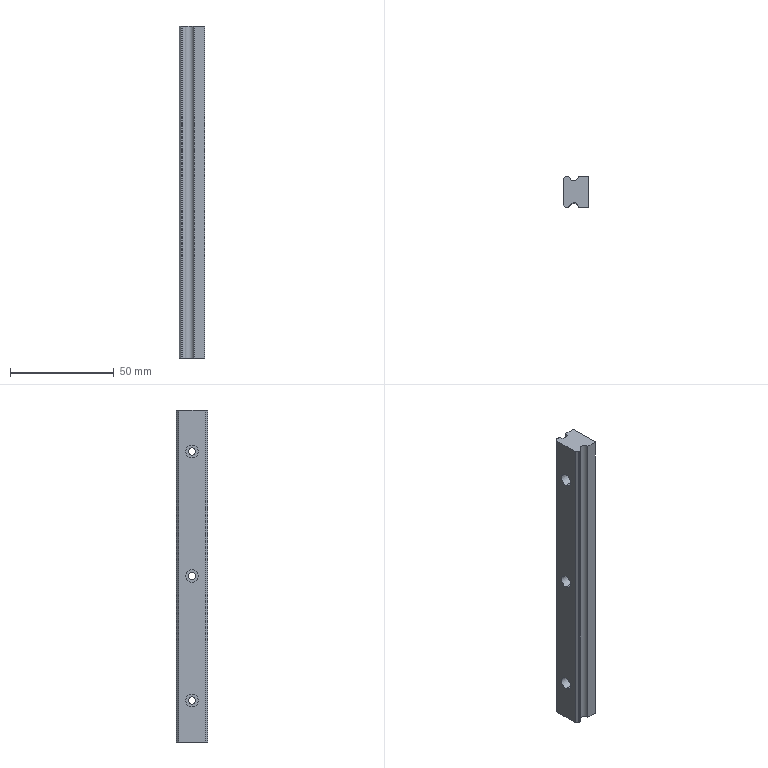Component | SolidWorks | SXRZ24_280-1_LinearGuide-1 | 1 solid | 30 faces | box 12.5 x 15 x 160 mm | volume 26679 mm3 | cylinder 17 | plane 13 | commonest cylinder face diameters 3.5 x6 6 x6 4.4 x3 3 x2
build123d program:
from build123d import *

# Parameters (mm, degrees)
BOSS_EXTRUDE1_DEPTH      = 140
BOSS_EXTRUDE1_DEPTH_BACK = 140
SKETCH7_W                = 125.064
SKETCH7_H                = 80
SKETCH7_W_2              = 316.061
SKETCH7_H_2              = 143.379
CUT_EXTRUDE1_DEPTH       = 141.757


with BuildPart() as part:
    # Sketch1 → Boss-Extrude1 (new, two sides: drawn at the far end of the back side and taken through both)
    with BuildSketch(Plane.XY.offset(-BOSS_EXTRUDE1_DEPTH_BACK)):
        with BuildLine():
            Line((-7.5, 0), (7.5, 0))
            Line((7.5, 0), (7.5, 5.105))
            ThreePointArc((7.5, 5.105), (5.348, 6.849), (6.608, 9.316))
            ThreePointArc((6.608, 9.316), (7.257, 9.869), (7.5, 10.687))
            Line((7.5, 10.687), (7.5, 11.376))
            Line((7.5, 11.376), (6.376, 12.5))
            Line((6.376, 12.5), (-6.376, 12.5))
            Line((-6.376, 12.5), (-7.5, 11.376))
            Line((-7.5, 11.376), (-7.5, 10.687))
            ThreePointArc((-7.5, 10.687), (-7.257, 9.869), (-6.608, 9.316))
            ThreePointArc((-6.608, 9.316), (-5.348, 6.849), (-7.5, 5.105))
            Line((-7.5, 5.105), (-7.5, 0))
        make_face()
    extrude(amount=BOSS_EXTRUDE1_DEPTH + BOSS_EXTRUDE1_DEPTH_BACK)

    # Sketch2 → Cut-Revolve1 (revolve, cut)
    with BuildSketch(Plane(origin=(0, 0, 0), x_dir=(0, 0, -1), z_dir=(1, 0, 0)), mode=Mode.PRIVATE) as cut_revolve1_sk:
        Polygon((120, 12.5), (123, 12.5), (123, 8), (121.75, 8), (121.75, 0), (120, 0), align=None)
    revolve(cut_revolve1_sk.sketch.rotate(Axis((0, 0, -120), (0, 1, 0)), 180), axis=Axis((0, 0, -120), (0, 1, 0)), mode=Mode.SUBTRACT)

    # Sketch3 → Cut-Revolve2 (revolve, cut)
    with BuildSketch(Plane(origin=(0, 0, 0), x_dir=(0, 0, -1), z_dir=(1, 0, 0)), mode=Mode.PRIVATE) as cut_revolve2_sk:
        Polygon((-120, 12.5), (-117, 12.5), (-117, 8), (-118.25, 8), (-118.25, 0), (-120, 0), align=None)
    revolve(cut_revolve2_sk.sketch.rotate(Axis((0, 0, 120), (0, 1, 0)), 180), axis=Axis((0, 0, 120), (0, 1, 0)), mode=Mode.SUBTRACT)

    # Sketch4 → Cut-Revolve3 (revolve, cut)
    with BuildSketch(Plane(origin=(0, 0, 0), x_dir=(0, 0, -1), z_dir=(1, 0, 0)), mode=Mode.PRIVATE) as cut_revolve3_sk:
        Polygon((-60, 12.5), (-57, 12.5), (-57, 8), (-58.25, 8), (-58.25, 0), (-60, 0), align=None)
    revolve(cut_revolve3_sk.sketch.rotate(Axis((0, 0, 60), (0, 1, 0)), 180), axis=Axis((0, 0, 60), (0, 1, 0)), mode=Mode.SUBTRACT)

    # Sketch5 → Cut-Revolve4 (revolve, cut)
    with BuildSketch(Plane(origin=(0, 0, 0), x_dir=(0, 0, -1), z_dir=(1, 0, 0)), mode=Mode.PRIVATE) as cut_revolve4_sk:
        Polygon((0, 12.5), (3, 12.5), (3, 8), (1.75, 8), (1.75, 0), (0, 0), align=None)
    revolve(cut_revolve4_sk.sketch.rotate(Axis((0, 0, 0), (0, 1, 0)), 180), axis=Axis((0, 0, 0), (0, 1, 0)), mode=Mode.SUBTRACT)

    # Sketch6 → Cut-Revolve5 (revolve, cut)
    with BuildSketch(Plane(origin=(0, 0, 0), x_dir=(0, 0, -1), z_dir=(1, 0, 0)), mode=Mode.PRIVATE) as cut_revolve5_sk:
        Polygon((60, 12.5), (63, 12.5), (63, 8), (61.75, 8), (61.75, 0), (60, 0), align=None)
    revolve(cut_revolve5_sk.sketch.rotate(Axis((0, 0, -60), (0, 1, 0)), 180), axis=Axis((0, 0, -60), (0, 1, 0)), mode=Mode.SUBTRACT)

    # Sketch7 → Cut-Extrude1 (cut, through all)
    with BuildSketch(Plane(origin=(0, 12.5, 0), x_dir=(1, 0, 0), z_dir=(0, 1, 0))):
        with Locations((-7.064, 120)):
            Rectangle(SKETCH7_W, SKETCH7_H)
        with Locations((6.803, -151.689)):
            Rectangle(SKETCH7_W_2, SKETCH7_H_2)
    extrude(amount=-CUT_EXTRUDE1_DEPTH, mode=Mode.SUBTRACT)


solid = part.part

# Placed as in the assembly
solid = solid.moved(Location((-772.135, -373.407, 1083.102), (0, 0, 90)))
STEP:
#1=COLOUR_RGB('',0.7922,0.8196,0.9333);
#2=FILL_AREA_STYLE_COLOUR('',#1);
#3=FILL_AREA_STYLE('',(#2));
#4=SURFACE_STYLE_FILL_AREA(#3);
#5=SURFACE_SIDE_STYLE('',(#4));
#6=SURFACE_STYLE_USAGE(.BOTH.,#5);
#7=PRESENTATION_STYLE_ASSIGNMENT((#6));
#8=CARTESIAN_POINT('',(-30.399,-14.701,40.211));
#9=VERTEX_POINT('',#8);
#10=CARTESIAN_POINT('',(-30.399,-14.701,40.349));
#11=VERTEX_POINT('',#10);
#12=CARTESIAN_POINT('',(-30.399,-14.701,40.28));
#13=DIRECTION('',(-1.,-0.,0.));
#14=DIRECTION('',(0.,0.,1.));
#15=AXIS2_PLACEMENT_3D('',#12,#13,#14);
#16=CIRCLE('',#15,0.0689);
#17=EDGE_CURVE('',#9,#11,#16,.T.);
#18=ORIENTED_EDGE('',*,*,#17,.F.);
#19=CARTESIAN_POINT('',(-30.714,-14.701,40.211));
#20=VERTEX_POINT('',#19);
#21=CARTESIAN_POINT('',(-30.399,-14.701,40.211));
#22=DIRECTION('',(-1.,-0.,0.));
#23=VECTOR('',#22,39.37);
#24=LINE('',#21,#23);
#25=EDGE_CURVE('',#9,#20,#24,.T.);
#26=ORIENTED_EDGE('',*,*,#25,.T.);
#27=CARTESIAN_POINT('',(-30.714,-14.701,40.349));
#28=VERTEX_POINT('',#27);
#29=CARTESIAN_POINT('',(-30.714,-14.701,40.28));
#30=DIRECTION('',(-1.,-0.,0.));
#31=DIRECTION('',(0.,0.,1.));
#32=AXIS2_PLACEMENT_3D('',#29,#30,#31);
#33=CIRCLE('',#32,0.0689);
#34=EDGE_CURVE('',#20,#28,#33,.T.);
#35=ORIENTED_EDGE('',*,*,#34,.T.);
#36=CARTESIAN_POINT('',(-30.399,-14.701,40.349));
#37=DIRECTION('',(-1.,-0.,0.));
#38=VECTOR('',#37,39.37);
#39=LINE('',#36,#38);
#40=EDGE_CURVE('',#11,#28,#39,.T.);
#41=ORIENTED_EDGE('',*,*,#40,.F.);
#42=EDGE_LOOP('',(#18,#26,#35,#41));
#43=FACE_OUTER_BOUND('',#42,.T.);
#44=CARTESIAN_POINT('',(-30.399,-14.701,40.28));
#45=DIRECTION('',(-1.,-0.,0.));
#46=DIRECTION('',(0.,0.,1.));
#47=AXIS2_PLACEMENT_3D('',#44,#45,#46);
#48=CYLINDRICAL_SURFACE('',#47,0.0689);
#49=ADVANCED_FACE('',(#43),#48,.F.);
#50=CARTESIAN_POINT('',(-30.714,-14.701,40.161));
#51=VERTEX_POINT('',#50);
#52=CARTESIAN_POINT('',(-30.714,-14.701,40.398));
#53=VERTEX_POINT('',#52);
#54=CARTESIAN_POINT('',(-30.714,-14.701,40.28));
#55=DIRECTION('',(-1.,-0.,0.));
#56=DIRECTION('',(0.,0.,1.));
#57=AXIS2_PLACEMENT_3D('',#54,#55,#56);
#58=CIRCLE('',#57,0.1181);
#59=EDGE_CURVE('',#51,#53,#58,.T.);
#60=ORIENTED_EDGE('',*,*,#59,.F.);
#61=CARTESIAN_POINT('',(-30.891,-14.701,40.161));
#62=VERTEX_POINT('',#61);
#63=CARTESIAN_POINT('',(-30.399,-14.701,40.161));
#64=DIRECTION('',(-1.,-0.,0.));
#65=VECTOR('',#64,39.37);
#66=LINE('',#63,#65);
#67=EDGE_CURVE('',#51,#62,#66,.T.);
#68=ORIENTED_EDGE('',*,*,#67,.T.);
#69=CARTESIAN_POINT('',(-30.891,-14.701,40.398));
#70=VERTEX_POINT('',#69);
#71=CARTESIAN_POINT('',(-30.891,-14.701,40.28));
#72=DIRECTION('',(-1.,-0.,0.));
#73=DIRECTION('',(0.,0.,1.));
#74=AXIS2_PLACEMENT_3D('',#71,#72,#73);
#75=CIRCLE('',#74,0.1181);
#76=EDGE_CURVE('',#62,#70,#75,.T.);
#77=ORIENTED_EDGE('',*,*,#76,.T.);
#78=CARTESIAN_POINT('',(-30.399,-14.701,40.398));
#79=DIRECTION('',(-1.,-0.,0.));
#80=VECTOR('',#79,39.37);
#81=LINE('',#78,#80);
#82=EDGE_CURVE('',#53,#70,#81,.T.);
#83=ORIENTED_EDGE('',*,*,#82,.F.);
#84=EDGE_LOOP('',(#60,#68,#77,#83));
#85=FACE_OUTER_BOUND('',#84,.T.);
#86=CARTESIAN_POINT('',(-30.399,-14.701,40.28));
#87=DIRECTION('',(-1.,-0.,0.));
#88=DIRECTION('',(0.,0.,1.));
#89=AXIS2_PLACEMENT_3D('',#86,#87,#88);
#90=CYLINDRICAL_SURFACE('',#89,0.1181);
#91=ADVANCED_FACE('',(#85),#90,.F.);
#92=CARTESIAN_POINT('',(-30.399,-14.701,42.573));
#93=VERTEX_POINT('',#92);
#94=CARTESIAN_POINT('',(-30.399,-14.701,42.711));
#95=VERTEX_POINT('',#94);
#96=CARTESIAN_POINT('',(-30.399,-14.701,42.642));
#97=DIRECTION('',(-1.,-0.,0.));
#98=DIRECTION('',(0.,0.,1.));
#99=AXIS2_PLACEMENT_3D('',#96,#97,#98);
#100=CIRCLE('',#99,0.0689);
#101=EDGE_CURVE('',#93,#95,#100,.T.);
#102=ORIENTED_EDGE('',*,*,#101,.F.);
#103=CARTESIAN_POINT('',(-30.714,-14.701,42.573));
#104=VERTEX_POINT('',#103);
#105=CARTESIAN_POINT('',(-30.399,-14.701,42.573));
#106=DIRECTION('',(-1.,-0.,0.));
#107=VECTOR('',#106,39.37);
#108=LINE('',#105,#107);
#109=EDGE_CURVE('',#93,#104,#108,.T.);
#110=ORIENTED_EDGE('',*,*,#109,.T.);
#111=CARTESIAN_POINT('',(-30.714,-14.701,42.711));
#112=VERTEX_POINT('',#111);
#113=CARTESIAN_POINT('',(-30.714,-14.701,42.642));
#114=DIRECTION('',(-1.,-0.,0.));
#115=DIRECTION('',(0.,0.,1.));
#116=AXIS2_PLACEMENT_3D('',#113,#114,#115);
#117=CIRCLE('',#116,0.0689);
#118=EDGE_CURVE('',#104,#112,#117,.T.);
#119=ORIENTED_EDGE('',*,*,#118,.T.);
#120=CARTESIAN_POINT('',(-30.399,-14.701,42.711));
#121=DIRECTION('',(-1.,-0.,0.));
#122=VECTOR('',#121,39.37);
#123=LINE('',#120,#122);
#124=EDGE_CURVE('',#95,#112,#123,.T.);
#125=ORIENTED_EDGE('',*,*,#124,.F.);
#126=EDGE_LOOP('',(#102,#110,#119,#125));
#127=FACE_OUTER_BOUND('',#126,.T.);
#128=CARTESIAN_POINT('',(-30.399,-14.701,42.642));
#129=DIRECTION('',(-1.,-0.,0.));
#130=DIRECTION('',(0.,0.,1.));
#131=AXIS2_PLACEMENT_3D('',#128,#129,#130);
#132=CYLINDRICAL_SURFACE('',#131,0.0689);
#133=ADVANCED_FACE('',(#127),#132,.F.);
#134=CARTESIAN_POINT('',(-30.714,-14.701,42.524));
#135=VERTEX_POINT('',#134);
#136=CARTESIAN_POINT('',(-30.714,-14.701,42.76));
#137=VERTEX_POINT('',#136);
#138=CARTESIAN_POINT('',(-30.714,-14.701,42.642));
#139=DIRECTION('',(-1.,-0.,0.));
#140=DIRECTION('',(0.,0.,1.));
#141=AXIS2_PLACEMENT_3D('',#138,#139,#140);
#142=CIRCLE('',#141,0.1181);
#143=EDGE_CURVE('',#135,#137,#142,.T.);
#144=ORIENTED_EDGE('',*,*,#143,.F.);
#145=CARTESIAN_POINT('',(-30.891,-14.701,42.524));
#146=VERTEX_POINT('',#145);
#147=CARTESIAN_POINT('',(-30.399,-14.701,42.524));
#148=DIRECTION('',(-1.,-0.,0.));
#149=VECTOR('',#148,39.37);
#150=LINE('',#147,#149);
#151=EDGE_CURVE('',#135,#146,#150,.T.);
#152=ORIENTED_EDGE('',*,*,#151,.T.);
#153=CARTESIAN_POINT('',(-30.891,-14.701,42.76));
#154=VERTEX_POINT('',#153);
#155=CARTESIAN_POINT('',(-30.891,-14.701,42.642));
#156=DIRECTION('',(-1.,-0.,0.));
#157=DIRECTION('',(0.,0.,1.));
#158=AXIS2_PLACEMENT_3D('',#155,#156,#157);
#159=CIRCLE('',#158,0.1181);
#160=EDGE_CURVE('',#146,#154,#159,.T.);
#161=ORIENTED_EDGE('',*,*,#160,.T.);
#162=CARTESIAN_POINT('',(-30.399,-14.701,42.76));
#163=DIRECTION('',(-1.,-0.,0.));
#164=VECTOR('',#163,39.37);
#165=LINE('',#162,#164);
#166=EDGE_CURVE('',#137,#154,#165,.T.);
#167=ORIENTED_EDGE('',*,*,#166,.F.);
#168=EDGE_LOOP('',(#144,#152,#161,#167));
#169=FACE_OUTER_BOUND('',#168,.T.);
#170=CARTESIAN_POINT('',(-30.399,-14.701,42.642));
#171=DIRECTION('',(-1.,-0.,0.));
#172=DIRECTION('',(0.,0.,1.));
#173=AXIS2_PLACEMENT_3D('',#170,#171,#172);
#174=CYLINDRICAL_SURFACE('',#173,0.1181);
#175=ADVANCED_FACE('',(#169),#174,.F.);
#176=CARTESIAN_POINT('',(-30.399,-14.701,44.935));
#177=VERTEX_POINT('',#176);
#178=CARTESIAN_POINT('',(-30.399,-14.701,45.073));
#179=VERTEX_POINT('',#178);
#180=CARTESIAN_POINT('',(-30.399,-14.701,45.004));
#181=DIRECTION('',(-1.,-0.,0.));
#182=DIRECTION('',(0.,0.,1.));
#183=AXIS2_PLACEMENT_3D('',#180,#181,#182);
#184=CIRCLE('',#183,0.0689);
#185=EDGE_CURVE('',#177,#179,#184,.T.);
#186=ORIENTED_EDGE('',*,*,#185,.F.);
#187=CARTESIAN_POINT('',(-30.714,-14.701,44.935));
#188=VERTEX_POINT('',#187);
#189=CARTESIAN_POINT('',(-30.399,-14.701,44.935));
#190=DIRECTION('',(-1.,-0.,0.));
#191=VECTOR('',#190,39.37);
#192=LINE('',#189,#191);
#193=EDGE_CURVE('',#177,#188,#192,.T.);
#194=ORIENTED_EDGE('',*,*,#193,.T.);
#195=CARTESIAN_POINT('',(-30.714,-14.701,45.073));
#196=VERTEX_POINT('',#195);
#197=CARTESIAN_POINT('',(-30.714,-14.701,45.004));
#198=DIRECTION('',(-1.,-0.,0.));
#199=DIRECTION('',(0.,0.,1.));
#200=AXIS2_PLACEMENT_3D('',#197,#198,#199);
#201=CIRCLE('',#200,0.0689);
#202=EDGE_CURVE('',#188,#196,#201,.T.);
#203=ORIENTED_EDGE('',*,*,#202,.T.);
#204=CARTESIAN_POINT('',(-30.399,-14.701,45.073));
#205=DIRECTION('',(-1.,-0.,0.));
#206=VECTOR('',#205,39.37);
#207=LINE('',#204,#206);
#208=EDGE_CURVE('',#179,#196,#207,.T.);
#209=ORIENTED_EDGE('',*,*,#208,.F.);
#210=EDGE_LOOP('',(#186,#194,#203,#209));
#211=FACE_OUTER_BOUND('',#210,.T.);
#212=CARTESIAN_POINT('',(-30.399,-14.701,45.004));
#213=DIRECTION('',(-1.,-0.,0.));
#214=DIRECTION('',(0.,0.,1.));
#215=AXIS2_PLACEMENT_3D('',#212,#213,#214);
#216=CYLINDRICAL_SURFACE('',#215,0.0689);
#217=ADVANCED_FACE('',(#211),#216,.F.);
#218=CARTESIAN_POINT('',(-30.714,-14.701,44.886));
#219=VERTEX_POINT('',#218);
#220=CARTESIAN_POINT('',(-30.714,-14.701,45.122));
#221=VERTEX_POINT('',#220);
#222=CARTESIAN_POINT('',(-30.714,-14.701,45.004));
#223=DIRECTION('',(-1.,-0.,0.));
#224=DIRECTION('',(0.,0.,1.));
#225=AXIS2_PLACEMENT_3D('',#222,#223,#224);
#226=CIRCLE('',#225,0.1181);
#227=EDGE_CURVE('',#219,#221,#226,.T.);
#228=ORIENTED_EDGE('',*,*,#227,.F.);
#229=CARTESIAN_POINT('',(-30.891,-14.701,44.886));
#230=VERTEX_POINT('',#229);
#231=CARTESIAN_POINT('',(-30.399,-14.701,44.886));
#232=DIRECTION('',(-1.,-0.,0.));
#233=VECTOR('',#232,39.37);
#234=LINE('',#231,#233);
#235=EDGE_CURVE('',#219,#230,#234,.T.);
#236=ORIENTED_EDGE('',*,*,#235,.T.);
#237=CARTESIAN_POINT('',(-30.891,-14.701,45.122));
#238=VERTEX_POINT('',#237);
#239=CARTESIAN_POINT('',(-30.891,-14.701,45.004));
#240=DIRECTION('',(-1.,-0.,0.));
#241=DIRECTION('',(0.,0.,1.));
#242=AXIS2_PLACEMENT_3D('',#239,#240,#241);
#243=CIRCLE('',#242,0.1181);
#244=EDGE_CURVE('',#230,#238,#243,.T.);
#245=ORIENTED_EDGE('',*,*,#244,.T.);
#246=CARTESIAN_POINT('',(-30.399,-14.701,45.122));
#247=DIRECTION('',(-1.,-0.,0.));
#248=VECTOR('',#247,39.37);
#249=LINE('',#246,#248);
#250=EDGE_CURVE('',#221,#238,#249,.T.);
#251=ORIENTED_EDGE('',*,*,#250,.F.);
#252=EDGE_LOOP('',(#228,#236,#245,#251));
#253=FACE_OUTER_BOUND('',#252,.T.);
#254=CARTESIAN_POINT('',(-30.399,-14.701,45.004));
#255=DIRECTION('',(-1.,-0.,0.));
#256=DIRECTION('',(0.,0.,1.));
#257=AXIS2_PLACEMENT_3D('',#254,#255,#256);
#258=CYLINDRICAL_SURFACE('',#257,0.1181);
#259=ADVANCED_FACE('',(#253),#258,.F.);
#260=CARTESIAN_POINT('',(-30.766,-14.441,45.791));
#261=VERTEX_POINT('',#260);
#262=CARTESIAN_POINT('',(-30.687,-14.492,45.791));
#263=VERTEX_POINT('',#262);
#264=CARTESIAN_POINT('',(-30.687,-14.406,45.791));
#265=DIRECTION('',(0.,-0.,1.));
#266=DIRECTION('',(0.,-1.,0.));
#267=AXIS2_PLACEMENT_3D('',#264,#265,#266);
#268=CIRCLE('',#267,0.08661);
#269=EDGE_CURVE('',#261,#263,#268,.T.);
#270=ORIENTED_EDGE('',*,*,#269,.T.);
#271=CARTESIAN_POINT('',(-30.687,-14.492,39.492));
#272=VERTEX_POINT('',#271);
#273=CARTESIAN_POINT('',(-30.687,-14.492,48.154));
#274=DIRECTION('',(-0.,0.,-1.));
#275=VECTOR('',#274,39.37);
#276=LINE('',#273,#275);
#277=EDGE_CURVE('',#263,#272,#276,.T.);
#278=ORIENTED_EDGE('',*,*,#277,.T.);
#279=CARTESIAN_POINT('',(-30.766,-14.441,39.492));
#280=VERTEX_POINT('',#279);
#281=CARTESIAN_POINT('',(-30.687,-14.406,39.492));
#282=DIRECTION('',(-0.,0.,-1.));
#283=DIRECTION('',(0.,1.,0.));
#284=AXIS2_PLACEMENT_3D('',#281,#282,#283);
#285=CIRCLE('',#284,0.08661);
#286=EDGE_CURVE('',#272,#280,#285,.T.);
#287=ORIENTED_EDGE('',*,*,#286,.T.);
#288=CARTESIAN_POINT('',(-30.766,-14.441,48.154));
#289=DIRECTION('',(-0.,0.,-1.));
#290=VECTOR('',#289,39.37);
#291=LINE('',#288,#290);
#292=EDGE_CURVE('',#261,#280,#291,.T.);
#293=ORIENTED_EDGE('',*,*,#292,.F.);
#294=EDGE_LOOP('',(#270,#278,#287,#293));
#295=FACE_OUTER_BOUND('',#294,.T.);
#296=CARTESIAN_POINT('',(-30.687,-14.406,48.154));
#297=DIRECTION('',(-0.,0.,-1.));
#298=DIRECTION('',(0.,-1.,0.));
#299=AXIS2_PLACEMENT_3D('',#296,#297,#298);
#300=CYLINDRICAL_SURFACE('',#299,0.08661);
#301=ADVANCED_FACE('',(#295),#300,.F.);
#302=CARTESIAN_POINT('',(-30.399,-14.701,42.642));
#303=DIRECTION('',(-1.,-0.,0.));
#304=DIRECTION('',(0.,0.,1.));
#305=AXIS2_PLACEMENT_3D('',#302,#303,#304);
#306=CIRCLE('',#305,0.0689);
#307=EDGE_CURVE('',#95,#93,#306,.T.);
#308=ORIENTED_EDGE('',*,*,#307,.T.);
#309=ORIENTED_EDGE('',*,*,#101,.T.);
#310=EDGE_LOOP('',(#308,#309));
#311=FACE_BOUND('',#310,.T.);
#312=CARTESIAN_POINT('',(-30.399,-14.406,45.791));
#313=VERTEX_POINT('',#312);
#314=CARTESIAN_POINT('',(-30.399,-14.406,39.492));
#315=VERTEX_POINT('',#314);
#316=CARTESIAN_POINT('',(-30.399,-14.406,48.154));
#317=DIRECTION('',(-0.,0.,-1.));
#318=VECTOR('',#317,39.37);
#319=LINE('',#316,#318);
#320=EDGE_CURVE('',#313,#315,#319,.T.);
#321=ORIENTED_EDGE('',*,*,#320,.F.);
#322=CARTESIAN_POINT('',(-30.399,-14.996,45.791));
#323=VERTEX_POINT('',#322);
#324=CARTESIAN_POINT('',(-30.399,-20.655,45.791));
#325=DIRECTION('',(0.,-1.,-0.));
#326=VECTOR('',#325,39.37);
#327=LINE('',#324,#326);
#328=EDGE_CURVE('',#313,#323,#327,.T.);
#329=ORIENTED_EDGE('',*,*,#328,.T.);
#330=CARTESIAN_POINT('',(-30.399,-14.996,39.492));
#331=VERTEX_POINT('',#330);
#332=CARTESIAN_POINT('',(-30.399,-14.996,48.154));
#333=DIRECTION('',(-0.,0.,-1.));
#334=VECTOR('',#333,39.37);
#335=LINE('',#332,#334);
#336=EDGE_CURVE('',#323,#331,#335,.T.);
#337=ORIENTED_EDGE('',*,*,#336,.T.);
#338=CARTESIAN_POINT('',(-30.399,-17.441,39.492));
#339=DIRECTION('',(-0.,1.,0.));
#340=VECTOR('',#339,39.37);
#341=LINE('',#338,#340);
#342=EDGE_CURVE('',#331,#315,#341,.T.);
#343=ORIENTED_EDGE('',*,*,#342,.T.);
#344=EDGE_LOOP('',(#321,#329,#337,#343));
#345=FACE_OUTER_BOUND('',#344,.T.);
#346=CARTESIAN_POINT('',(-30.399,-14.701,45.004));
#347=DIRECTION('',(-1.,-0.,0.));
#348=DIRECTION('',(0.,0.,1.));
#349=AXIS2_PLACEMENT_3D('',#346,#347,#348);
#350=CIRCLE('',#349,0.0689);
#351=EDGE_CURVE('',#179,#177,#350,.T.);
#352=ORIENTED_EDGE('',*,*,#351,.T.);
#353=ORIENTED_EDGE('',*,*,#185,.T.);
#354=EDGE_LOOP('',(#352,#353));
#355=FACE_BOUND('',#354,.T.);
#356=CARTESIAN_POINT('',(-30.399,-14.701,40.28));
#357=DIRECTION('',(-1.,-0.,0.));
#358=DIRECTION('',(0.,0.,1.));
#359=AXIS2_PLACEMENT_3D('',#356,#357,#358);
#360=CIRCLE('',#359,0.0689);
#361=EDGE_CURVE('',#11,#9,#360,.T.);
#362=ORIENTED_EDGE('',*,*,#361,.T.);
#363=ORIENTED_EDGE('',*,*,#17,.T.);
#364=EDGE_LOOP('',(#362,#363));
#365=FACE_BOUND('',#364,.T.);
#366=CARTESIAN_POINT('',(-30.399,-14.996,48.154));
#367=DIRECTION('',(-1.,-0.,0.));
#368=DIRECTION('',(0.,-0.,1.));
#369=AXIS2_PLACEMENT_3D('',#366,#367,#368);
#370=PLANE('',#369);
#371=ADVANCED_FACE('',(#311,#345,#355,#365),#370,.F.);
#372=CARTESIAN_POINT('',(-30.891,-14.701,42.642));
#373=DIRECTION('',(-1.,-0.,0.));
#374=DIRECTION('',(0.,0.,1.));
#375=AXIS2_PLACEMENT_3D('',#372,#373,#374);
#376=CIRCLE('',#375,0.1181);
#377=EDGE_CURVE('',#154,#146,#376,.T.);
#378=ORIENTED_EDGE('',*,*,#377,.F.);
#379=ORIENTED_EDGE('',*,*,#160,.F.);
#380=EDGE_LOOP('',(#378,#379));
#381=FACE_BOUND('',#380,.T.);
#382=CARTESIAN_POINT('',(-30.891,-14.952,45.791));
#383=VERTEX_POINT('',#382);
#384=CARTESIAN_POINT('',(-30.891,-14.952,39.492));
#385=VERTEX_POINT('',#384);
#386=CARTESIAN_POINT('',(-30.891,-14.952,48.154));
#387=DIRECTION('',(-0.,0.,-1.));
#388=VECTOR('',#387,39.37);
#389=LINE('',#386,#388);
#390=EDGE_CURVE('',#383,#385,#389,.T.);
#391=ORIENTED_EDGE('',*,*,#390,.F.);
#392=CARTESIAN_POINT('',(-30.891,-14.45,45.791));
#393=VERTEX_POINT('',#392);
#394=CARTESIAN_POINT('',(-30.891,-20.655,45.791));
#395=DIRECTION('',(0.,-1.,-0.));
#396=VECTOR('',#395,39.37);
#397=LINE('',#394,#396);
#398=EDGE_CURVE('',#393,#383,#397,.T.);
#399=ORIENTED_EDGE('',*,*,#398,.F.);
#400=CARTESIAN_POINT('',(-30.891,-14.45,39.492));
#401=VERTEX_POINT('',#400);
#402=CARTESIAN_POINT('',(-30.891,-14.45,48.154));
#403=DIRECTION('',(-0.,0.,-1.));
#404=VECTOR('',#403,39.37);
#405=LINE('',#402,#404);
#406=EDGE_CURVE('',#393,#401,#405,.T.);
#407=ORIENTED_EDGE('',*,*,#406,.T.);
#408=CARTESIAN_POINT('',(-30.891,-17.441,39.492));
#409=DIRECTION('',(-0.,1.,0.));
#410=VECTOR('',#409,39.37);
#411=LINE('',#408,#410);
#412=EDGE_CURVE('',#385,#401,#411,.T.);
#413=ORIENTED_EDGE('',*,*,#412,.F.);
#414=EDGE_LOOP('',(#391,#399,#407,#413));
#415=FACE_OUTER_BOUND('',#414,.T.);
#416=CARTESIAN_POINT('',(-30.891,-14.701,45.004));
#417=DIRECTION('',(-1.,-0.,0.));
#418=DIRECTION('',(0.,0.,1.));
#419=AXIS2_PLACEMENT_3D('',#416,#417,#418);
#420=CIRCLE('',#419,0.1181);
#421=EDGE_CURVE('',#238,#230,#420,.T.);
#422=ORIENTED_EDGE('',*,*,#421,.F.);
#423=ORIENTED_EDGE('',*,*,#244,.F.);
#424=EDGE_LOOP('',(#422,#423));
#425=FACE_BOUND('',#424,.T.);
#426=CARTESIAN_POINT('',(-30.891,-14.701,40.28));
#427=DIRECTION('',(-1.,-0.,0.));
#428=DIRECTION('',(0.,0.,1.));
#429=AXIS2_PLACEMENT_3D('',#426,#427,#428);
#430=CIRCLE('',#429,0.1181);
#431=EDGE_CURVE('',#70,#62,#430,.T.);
#432=ORIENTED_EDGE('',*,*,#431,.F.);
#433=ORIENTED_EDGE('',*,*,#76,.F.);
#434=EDGE_LOOP('',(#432,#433));
#435=FACE_BOUND('',#434,.T.);
#436=CARTESIAN_POINT('',(-30.891,-14.45,48.154));
#437=DIRECTION('',(1.,0.,-0.));
#438=DIRECTION('',(-0.,0.,-1.));
#439=AXIS2_PLACEMENT_3D('',#436,#437,#438);
#440=PLANE('',#439);
#441=ADVANCED_FACE('',(#381,#415,#425,#435),#440,.F.);
#442=ORIENTED_EDGE('',*,*,#336,.F.);
#443=CARTESIAN_POINT('',(-30.6,-14.996,45.791));
#444=VERTEX_POINT('',#443);
#445=CARTESIAN_POINT('',(-30.6,-14.996,45.791));
#446=DIRECTION('',(-1.,-0.,0.));
#447=VECTOR('',#446,39.37);
#448=LINE('',#445,#447);
#449=EDGE_CURVE('',#323,#444,#448,.T.);
#450=ORIENTED_EDGE('',*,*,#449,.T.);
#451=CARTESIAN_POINT('',(-30.6,-14.996,39.492));
#452=VERTEX_POINT('',#451);
#453=CARTESIAN_POINT('',(-30.6,-14.996,48.154));
#454=DIRECTION('',(-0.,0.,-1.));
#455=VECTOR('',#454,39.37);
#456=LINE('',#453,#455);
#457=EDGE_CURVE('',#444,#452,#456,.T.);
#458=ORIENTED_EDGE('',*,*,#457,.T.);
#459=CARTESIAN_POINT('',(-30.6,-14.996,39.492));
#460=DIRECTION('',(1.,0.,-0.));
#461=VECTOR('',#460,39.37);
#462=LINE('',#459,#461);
#463=EDGE_CURVE('',#452,#331,#462,.T.);
#464=ORIENTED_EDGE('',*,*,#463,.T.);
#465=EDGE_LOOP('',(#442,#450,#458,#464));
#466=FACE_OUTER_BOUND('',#465,.T.);
#467=CARTESIAN_POINT('',(-30.6,-14.996,48.154));
#468=DIRECTION('',(-0.,1.,0.));
#469=DIRECTION('',(-0.,0.,-1.));
#470=AXIS2_PLACEMENT_3D('',#467,#468,#469);
#471=PLANE('',#470);
#472=ADVANCED_FACE('',(#466),#471,.F.);
#473=CARTESIAN_POINT('',(-30.6,-14.406,45.791));
#474=VERTEX_POINT('',#473);
#475=CARTESIAN_POINT('',(-30.6,-14.406,39.492));
#476=VERTEX_POINT('',#475);
#477=CARTESIAN_POINT('',(-30.6,-14.406,48.154));
#478=DIRECTION('',(-0.,0.,-1.));
#479=VECTOR('',#478,39.37);
#480=LINE('',#477,#479);
#481=EDGE_CURVE('',#474,#476,#480,.T.);
#482=ORIENTED_EDGE('',*,*,#481,.F.);
#483=CARTESIAN_POINT('',(-30.399,-14.406,45.791));
#484=DIRECTION('',(1.,0.,-0.));
#485=VECTOR('',#484,39.37);
#486=LINE('',#483,#485);
#487=EDGE_CURVE('',#474,#313,#486,.T.);
#488=ORIENTED_EDGE('',*,*,#487,.T.);
#489=ORIENTED_EDGE('',*,*,#320,.T.);
#490=CARTESIAN_POINT('',(-30.399,-14.406,39.492));
#491=DIRECTION('',(-1.,-0.,0.));
#492=VECTOR('',#491,39.37);
#493=LINE('',#490,#492);
#494=EDGE_CURVE('',#315,#476,#493,.T.);
#495=ORIENTED_EDGE('',*,*,#494,.T.);
#496=EDGE_LOOP('',(#482,#488,#489,#495));
#497=FACE_OUTER_BOUND('',#496,.T.);
#498=CARTESIAN_POINT('',(-30.399,-14.406,48.154));
#499=DIRECTION('',(0.,-1.,-0.));
#500=DIRECTION('',(0.,-0.,1.));
#501=AXIS2_PLACEMENT_3D('',#498,#499,#500);
#502=PLANE('',#501);
#503=ADVANCED_FACE('',(#497),#502,.F.);
#504=ORIENTED_EDGE('',*,*,#277,.F.);
#505=CARTESIAN_POINT('',(-30.687,-14.406,45.791));
#506=DIRECTION('',(0.,-0.,1.));
#507=DIRECTION('',(0.,-1.,0.));
#508=AXIS2_PLACEMENT_3D('',#505,#506,#507);
#509=CIRCLE('',#508,0.08661);
#510=EDGE_CURVE('',#263,#474,#509,.T.);
#511=ORIENTED_EDGE('',*,*,#510,.T.);
#512=ORIENTED_EDGE('',*,*,#481,.T.);
#513=CARTESIAN_POINT('',(-30.687,-14.406,39.492));
#514=DIRECTION('',(-0.,0.,-1.));
#515=DIRECTION('',(0.,1.,0.));
#516=AXIS2_PLACEMENT_3D('',#513,#514,#515);
#517=CIRCLE('',#516,0.08661);
#518=EDGE_CURVE('',#476,#272,#517,.T.);
#519=ORIENTED_EDGE('',*,*,#518,.T.);
#520=EDGE_LOOP('',(#504,#511,#512,#519));
#521=FACE_OUTER_BOUND('',#520,.T.);
#522=CARTESIAN_POINT('',(-30.687,-14.406,48.154));
#523=DIRECTION('',(-0.,0.,-1.));
#524=DIRECTION('',(0.,-1.,0.));
#525=AXIS2_PLACEMENT_3D('',#522,#523,#524);
#526=CYLINDRICAL_SURFACE('',#525,0.08661);
#527=ADVANCED_FACE('',(#521),#526,.F.);
#528=CARTESIAN_POINT('',(-30.82,-14.406,45.791));
#529=VERTEX_POINT('',#528);
#530=CARTESIAN_POINT('',(-30.82,-14.406,39.492));
#531=VERTEX_POINT('',#530);
#532=CARTESIAN_POINT('',(-30.82,-14.406,48.154));
#533=DIRECTION('',(-0.,0.,-1.));
#534=VECTOR('',#533,39.37);
#535=LINE('',#532,#534);
#536=EDGE_CURVE('',#529,#531,#535,.T.);
#537=ORIENTED_EDGE('',*,*,#536,.F.);
#538=CARTESIAN_POINT('',(-30.82,-14.465,45.791));
#539=DIRECTION('',(-0.,0.,-1.));
#540=DIRECTION('',(0.,-1.,0.));
#541=AXIS2_PLACEMENT_3D('',#538,#539,#540);
#542=CIRCLE('',#541,0.05906);
#543=EDGE_CURVE('',#529,#261,#542,.T.);
#544=ORIENTED_EDGE('',*,*,#543,.T.);
#545=ORIENTED_EDGE('',*,*,#292,.T.);
#546=CARTESIAN_POINT('',(-30.82,-14.465,39.492));
#547=DIRECTION('',(0.,-0.,1.));
#548=DIRECTION('',(0.,1.,0.));
#549=AXIS2_PLACEMENT_3D('',#546,#547,#548);
#550=CIRCLE('',#549,0.05906);
#551=EDGE_CURVE('',#280,#531,#550,.T.);
#552=ORIENTED_EDGE('',*,*,#551,.T.);
#553=EDGE_LOOP('',(#537,#544,#545,#552));
#554=FACE_OUTER_BOUND('',#553,.T.);
#555=CARTESIAN_POINT('',(-30.82,-14.465,48.154));
#556=DIRECTION('',(-0.,0.,-1.));
#557=DIRECTION('',(0.,-1.,0.));
#558=AXIS2_PLACEMENT_3D('',#555,#556,#557);
#559=CYLINDRICAL_SURFACE('',#558,0.05906);
#560=ADVANCED_FACE('',(#554),#559,.T.);
#561=CARTESIAN_POINT('',(-30.847,-14.406,45.791));
#562=VERTEX_POINT('',#561);
#563=CARTESIAN_POINT('',(-30.847,-14.406,39.492));
#564=VERTEX_POINT('',#563);
#565=CARTESIAN_POINT('',(-30.847,-14.406,48.154));
#566=DIRECTION('',(-0.,0.,-1.));
#567=VECTOR('',#566,39.37);
#568=LINE('',#565,#567);
#569=EDGE_CURVE('',#562,#564,#568,.T.);
#570=ORIENTED_EDGE('',*,*,#569,.F.);
#571=CARTESIAN_POINT('',(-30.82,-14.406,45.791));
#572=DIRECTION('',(1.,0.,-0.));
#573=VECTOR('',#572,39.37);
#574=LINE('',#571,#573);
#575=EDGE_CURVE('',#562,#529,#574,.T.);
#576=ORIENTED_EDGE('',*,*,#575,.T.);
#577=ORIENTED_EDGE('',*,*,#536,.T.);
#578=CARTESIAN_POINT('',(-30.82,-14.406,39.492));
#579=DIRECTION('',(-1.,-0.,0.));
#580=VECTOR('',#579,39.37);
#581=LINE('',#578,#580);
#582=EDGE_CURVE('',#531,#564,#581,.T.);
#583=ORIENTED_EDGE('',*,*,#582,.T.);
#584=EDGE_LOOP('',(#570,#576,#577,#583));
#585=FACE_OUTER_BOUND('',#584,.T.);
#586=CARTESIAN_POINT('',(-30.82,-14.406,48.154));
#587=DIRECTION('',(0.,-1.,-0.));
#588=DIRECTION('',(0.,-0.,1.));
#589=AXIS2_PLACEMENT_3D('',#586,#587,#588);
#590=PLANE('',#589);
#591=ADVANCED_FACE('',(#585),#590,.F.);
#592=ORIENTED_EDGE('',*,*,#406,.F.);
#593=CARTESIAN_POINT('',(-30.847,-14.406,45.791));
#594=DIRECTION('',(0.7071,0.7071,0.));
#595=VECTOR('',#594,39.37);
#596=LINE('',#593,#595);
#597=EDGE_CURVE('',#393,#562,#596,.T.);
#598=ORIENTED_EDGE('',*,*,#597,.T.);
#599=ORIENTED_EDGE('',*,*,#569,.T.);
#600=CARTESIAN_POINT('',(-30.847,-14.406,39.492));
#601=DIRECTION('',(-0.7071,-0.7071,-0.));
#602=VECTOR('',#601,39.37);
#603=LINE('',#600,#602);
#604=EDGE_CURVE('',#564,#401,#603,.T.);
#605=ORIENTED_EDGE('',*,*,#604,.T.);
#606=EDGE_LOOP('',(#592,#598,#599,#605));
#607=FACE_OUTER_BOUND('',#606,.T.);
#608=CARTESIAN_POINT('',(-30.847,-14.406,48.154));
#609=DIRECTION('',(0.7071,-0.7071,-0.));
#610=DIRECTION('',(0.7071,0.7071,0.));
#611=AXIS2_PLACEMENT_3D('',#608,#609,#610);
#612=PLANE('',#611);
#613=ADVANCED_FACE('',(#607),#612,.F.);
#614=CARTESIAN_POINT('',(-30.847,-14.996,45.791));
#615=VERTEX_POINT('',#614);
#616=CARTESIAN_POINT('',(-30.847,-14.996,39.492));
#617=VERTEX_POINT('',#616);
#618=CARTESIAN_POINT('',(-30.847,-14.996,48.154));
#619=DIRECTION('',(-0.,0.,-1.));
#620=VECTOR('',#619,39.37);
#621=LINE('',#618,#620);
#622=EDGE_CURVE('',#615,#617,#621,.T.);
#623=ORIENTED_EDGE('',*,*,#622,.F.);
#624=CARTESIAN_POINT('',(-30.891,-14.952,45.791));
#625=DIRECTION('',(-0.7071,0.7071,0.));
#626=VECTOR('',#625,39.37);
#627=LINE('',#624,#626);
#628=EDGE_CURVE('',#615,#383,#627,.T.);
#629=ORIENTED_EDGE('',*,*,#628,.T.);
#630=ORIENTED_EDGE('',*,*,#390,.T.);
#631=CARTESIAN_POINT('',(-30.891,-14.952,39.492));
#632=DIRECTION('',(0.7071,-0.7071,-0.));
#633=VECTOR('',#632,39.37);
#634=LINE('',#631,#633);
#635=EDGE_CURVE('',#385,#617,#634,.T.);
#636=ORIENTED_EDGE('',*,*,#635,.T.);
#637=EDGE_LOOP('',(#623,#629,#630,#636));
#638=FACE_OUTER_BOUND('',#637,.T.);
#639=CARTESIAN_POINT('',(-30.891,-14.952,48.154));
#640=DIRECTION('',(0.7071,0.7071,0.));
#641=DIRECTION('',(-0.7071,0.7071,0.));
#642=AXIS2_PLACEMENT_3D('',#639,#640,#641);
#643=PLANE('',#642);
#644=ADVANCED_FACE('',(#638),#643,.F.);
#645=CARTESIAN_POINT('',(-30.82,-14.996,45.791));
#646=VERTEX_POINT('',#645);
#647=CARTESIAN_POINT('',(-30.82,-14.996,39.492));
#648=VERTEX_POINT('',#647);
#649=CARTESIAN_POINT('',(-30.82,-14.996,48.154));
#650=DIRECTION('',(-0.,0.,-1.));
#651=VECTOR('',#650,39.37);
#652=LINE('',#649,#651);
#653=EDGE_CURVE('',#646,#648,#652,.T.);
#654=ORIENTED_EDGE('',*,*,#653,.F.);
#655=CARTESIAN_POINT('',(-30.847,-14.996,45.791));
#656=DIRECTION('',(-1.,-0.,0.));
#657=VECTOR('',#656,39.37);
#658=LINE('',#655,#657);
#659=EDGE_CURVE('',#646,#615,#658,.T.);
#660=ORIENTED_EDGE('',*,*,#659,.T.);
#661=ORIENTED_EDGE('',*,*,#622,.T.);
#662=CARTESIAN_POINT('',(-30.847,-14.996,39.492));
#663=DIRECTION('',(1.,0.,-0.));
#664=VECTOR('',#663,39.37);
#665=LINE('',#662,#664);
#666=EDGE_CURVE('',#617,#648,#665,.T.);
#667=ORIENTED_EDGE('',*,*,#666,.T.);
#668=EDGE_LOOP('',(#654,#660,#661,#667));
#669=FACE_OUTER_BOUND('',#668,.T.);
#670=CARTESIAN_POINT('',(-30.847,-14.996,48.154));
#671=DIRECTION('',(-0.,1.,0.));
#672=DIRECTION('',(-0.,0.,-1.));
#673=AXIS2_PLACEMENT_3D('',#670,#671,#672);
#674=PLANE('',#673);
#675=ADVANCED_FACE('',(#669),#674,.F.);
#676=CARTESIAN_POINT('',(-30.766,-14.961,45.791));
#677=VERTEX_POINT('',#676);
#678=CARTESIAN_POINT('',(-30.766,-14.961,39.492));
#679=VERTEX_POINT('',#678);
#680=CARTESIAN_POINT('',(-30.766,-14.961,48.154));
#681=DIRECTION('',(-0.,0.,-1.));
#682=VECTOR('',#681,39.37);
#683=LINE('',#680,#682);
#684=EDGE_CURVE('',#677,#679,#683,.T.);
#685=ORIENTED_EDGE('',*,*,#684,.F.);
#686=CARTESIAN_POINT('',(-30.82,-14.937,45.791));
#687=DIRECTION('',(-0.,0.,-1.));
#688=DIRECTION('',(0.,-1.,0.));
#689=AXIS2_PLACEMENT_3D('',#686,#687,#688);
#690=CIRCLE('',#689,0.05906);
#691=EDGE_CURVE('',#677,#646,#690,.T.);
#692=ORIENTED_EDGE('',*,*,#691,.T.);
#693=ORIENTED_EDGE('',*,*,#653,.T.);
#694=CARTESIAN_POINT('',(-30.82,-14.937,39.492));
#695=DIRECTION('',(0.,-0.,1.));
#696=DIRECTION('',(0.,1.,0.));
#697=AXIS2_PLACEMENT_3D('',#694,#695,#696);
#698=CIRCLE('',#697,0.05906);
#699=EDGE_CURVE('',#648,#679,#698,.T.);
#700=ORIENTED_EDGE('',*,*,#699,.T.);
#701=EDGE_LOOP('',(#685,#692,#693,#700));
#702=FACE_OUTER_BOUND('',#701,.T.);
#703=CARTESIAN_POINT('',(-30.82,-14.937,48.154));
#704=DIRECTION('',(-0.,0.,-1.));
#705=DIRECTION('',(0.,-1.,0.));
#706=AXIS2_PLACEMENT_3D('',#703,#704,#705);
#707=CYLINDRICAL_SURFACE('',#706,0.05906);
#708=ADVANCED_FACE('',(#702),#707,.T.);
#709=ORIENTED_EDGE('',*,*,#457,.F.);
#710=CARTESIAN_POINT('',(-30.687,-14.996,45.791));
#711=DIRECTION('',(0.,-0.,1.));
#712=DIRECTION('',(0.,-1.,0.));
#713=AXIS2_PLACEMENT_3D('',#710,#711,#712);
#714=CIRCLE('',#713,0.08661);
#715=EDGE_CURVE('',#444,#677,#714,.T.);
#716=ORIENTED_EDGE('',*,*,#715,.T.);
#717=ORIENTED_EDGE('',*,*,#684,.T.);
#718=CARTESIAN_POINT('',(-30.687,-14.996,39.492));
#719=DIRECTION('',(-0.,0.,-1.));
#720=DIRECTION('',(0.,1.,0.));
#721=AXIS2_PLACEMENT_3D('',#718,#719,#720);
#722=CIRCLE('',#721,0.08661);
#723=EDGE_CURVE('',#679,#452,#722,.T.);
#724=ORIENTED_EDGE('',*,*,#723,.T.);
#725=EDGE_LOOP('',(#709,#716,#717,#724));
#726=FACE_OUTER_BOUND('',#725,.T.);
#727=CARTESIAN_POINT('',(-30.687,-14.996,48.154));
#728=DIRECTION('',(-0.,0.,-1.));
#729=DIRECTION('',(0.,-1.,0.));
#730=AXIS2_PLACEMENT_3D('',#727,#728,#729);
#731=CYLINDRICAL_SURFACE('',#730,0.08661);
#732=ADVANCED_FACE('',(#726),#731,.F.);
#733=ORIENTED_EDGE('',*,*,#235,.F.);
#734=CARTESIAN_POINT('',(-30.714,-14.701,45.004));
#735=DIRECTION('',(-1.,-0.,0.));
#736=DIRECTION('',(0.,0.,1.));
#737=AXIS2_PLACEMENT_3D('',#734,#735,#736);
#738=CIRCLE('',#737,0.1181);
#739=EDGE_CURVE('',#221,#219,#738,.T.);
#740=ORIENTED_EDGE('',*,*,#739,.F.);
#741=ORIENTED_EDGE('',*,*,#250,.T.);
#742=ORIENTED_EDGE('',*,*,#421,.T.);
#743=EDGE_LOOP('',(#733,#740,#741,#742));
#744=FACE_OUTER_BOUND('',#743,.T.);
#745=CARTESIAN_POINT('',(-30.399,-14.701,45.004));
#746=DIRECTION('',(-1.,-0.,0.));
#747=DIRECTION('',(0.,0.,1.));
#748=AXIS2_PLACEMENT_3D('',#745,#746,#747);
#749=CYLINDRICAL_SURFACE('',#748,0.1181);
#750=ADVANCED_FACE('',(#744),#749,.F.);
#751=ORIENTED_EDGE('',*,*,#739,.T.);
#752=ORIENTED_EDGE('',*,*,#227,.T.);
#753=EDGE_LOOP('',(#751,#752));
#754=FACE_OUTER_BOUND('',#753,.T.);
#755=CARTESIAN_POINT('',(-30.714,-14.701,45.004));
#756=DIRECTION('',(-1.,-0.,0.));
#757=DIRECTION('',(0.,0.,1.));
#758=AXIS2_PLACEMENT_3D('',#755,#756,#757);
#759=CIRCLE('',#758,0.0689);
#760=EDGE_CURVE('',#196,#188,#759,.T.);
#761=ORIENTED_EDGE('',*,*,#760,.F.);
#762=ORIENTED_EDGE('',*,*,#202,.F.);
#763=EDGE_LOOP('',(#761,#762));
#764=FACE_BOUND('',#763,.T.);
#765=CARTESIAN_POINT('',(-30.714,-14.701,44.886));
#766=DIRECTION('',(-1.,-0.,0.));
#767=DIRECTION('',(0.,-0.,1.));
#768=AXIS2_PLACEMENT_3D('',#765,#766,#767);
#769=PLANE('',#768);
#770=ADVANCED_FACE('',(#754,#764),#769,.T.);
#771=ORIENTED_EDGE('',*,*,#193,.F.);
#772=ORIENTED_EDGE('',*,*,#351,.F.);
#773=ORIENTED_EDGE('',*,*,#208,.T.);
#774=ORIENTED_EDGE('',*,*,#760,.T.);
#775=EDGE_LOOP('',(#771,#772,#773,#774));
#776=FACE_OUTER_BOUND('',#775,.T.);
#777=CARTESIAN_POINT('',(-30.399,-14.701,45.004));
#778=DIRECTION('',(-1.,-0.,0.));
#779=DIRECTION('',(0.,0.,1.));
#780=AXIS2_PLACEMENT_3D('',#777,#778,#779);
#781=CYLINDRICAL_SURFACE('',#780,0.0689);
#782=ADVANCED_FACE('',(#776),#781,.F.);
#783=ORIENTED_EDGE('',*,*,#151,.F.);
#784=CARTESIAN_POINT('',(-30.714,-14.701,42.642));
#785=DIRECTION('',(-1.,-0.,0.));
#786=DIRECTION('',(0.,0.,1.));
#787=AXIS2_PLACEMENT_3D('',#784,#785,#786);
#788=CIRCLE('',#787,0.1181);
#789=EDGE_CURVE('',#137,#135,#788,.T.);
#790=ORIENTED_EDGE('',*,*,#789,.F.);
#791=ORIENTED_EDGE('',*,*,#166,.T.);
#792=ORIENTED_EDGE('',*,*,#377,.T.);
#793=EDGE_LOOP('',(#783,#790,#791,#792));
#794=FACE_OUTER_BOUND('',#793,.T.);
#795=CARTESIAN_POINT('',(-30.399,-14.701,42.642));
#796=DIRECTION('',(-1.,-0.,0.));
#797=DIRECTION('',(0.,0.,1.));
#798=AXIS2_PLACEMENT_3D('',#795,#796,#797);
#799=CYLINDRICAL_SURFACE('',#798,0.1181);
#800=ADVANCED_FACE('',(#794),#799,.F.);
#801=ORIENTED_EDGE('',*,*,#789,.T.);
#802=ORIENTED_EDGE('',*,*,#143,.T.);
#803=EDGE_LOOP('',(#801,#802));
#804=FACE_OUTER_BOUND('',#803,.T.);
#805=CARTESIAN_POINT('',(-30.714,-14.701,42.642));
#806=DIRECTION('',(-1.,-0.,0.));
#807=DIRECTION('',(0.,0.,1.));
#808=AXIS2_PLACEMENT_3D('',#805,#806,#807);
#809=CIRCLE('',#808,0.0689);
#810=EDGE_CURVE('',#112,#104,#809,.T.);
#811=ORIENTED_EDGE('',*,*,#810,.F.);
#812=ORIENTED_EDGE('',*,*,#118,.F.);
#813=EDGE_LOOP('',(#811,#812));
#814=FACE_BOUND('',#813,.T.);
#815=CARTESIAN_POINT('',(-30.714,-14.701,42.524));
#816=DIRECTION('',(-1.,-0.,0.));
#817=DIRECTION('',(0.,-0.,1.));
#818=AXIS2_PLACEMENT_3D('',#815,#816,#817);
#819=PLANE('',#818);
#820=ADVANCED_FACE('',(#804,#814),#819,.T.);
#821=ORIENTED_EDGE('',*,*,#109,.F.);
#822=ORIENTED_EDGE('',*,*,#307,.F.);
#823=ORIENTED_EDGE('',*,*,#124,.T.);
#824=ORIENTED_EDGE('',*,*,#810,.T.);
#825=EDGE_LOOP('',(#821,#822,#823,#824));
#826=FACE_OUTER_BOUND('',#825,.T.);
#827=CARTESIAN_POINT('',(-30.399,-14.701,42.642));
#828=DIRECTION('',(-1.,-0.,0.));
#829=DIRECTION('',(0.,0.,1.));
#830=AXIS2_PLACEMENT_3D('',#827,#828,#829);
#831=CYLINDRICAL_SURFACE('',#830,0.0689);
#832=ADVANCED_FACE('',(#826),#831,.F.);
#833=ORIENTED_EDGE('',*,*,#67,.F.);
#834=CARTESIAN_POINT('',(-30.714,-14.701,40.28));
#835=DIRECTION('',(-1.,-0.,0.));
#836=DIRECTION('',(0.,0.,1.));
#837=AXIS2_PLACEMENT_3D('',#834,#835,#836);
#838=CIRCLE('',#837,0.1181);
#839=EDGE_CURVE('',#53,#51,#838,.T.);
#840=ORIENTED_EDGE('',*,*,#839,.F.);
#841=ORIENTED_EDGE('',*,*,#82,.T.);
#842=ORIENTED_EDGE('',*,*,#431,.T.);
#843=EDGE_LOOP('',(#833,#840,#841,#842));
#844=FACE_OUTER_BOUND('',#843,.T.);
#845=CARTESIAN_POINT('',(-30.399,-14.701,40.28));
#846=DIRECTION('',(-1.,-0.,0.));
#847=DIRECTION('',(0.,0.,1.));
#848=AXIS2_PLACEMENT_3D('',#845,#846,#847);
#849=CYLINDRICAL_SURFACE('',#848,0.1181);
#850=ADVANCED_FACE('',(#844),#849,.F.);
#851=ORIENTED_EDGE('',*,*,#839,.T.);
#852=ORIENTED_EDGE('',*,*,#59,.T.);
#853=EDGE_LOOP('',(#851,#852));
#854=FACE_OUTER_BOUND('',#853,.T.);
#855=CARTESIAN_POINT('',(-30.714,-14.701,40.28));
#856=DIRECTION('',(-1.,-0.,0.));
#857=DIRECTION('',(0.,0.,1.));
#858=AXIS2_PLACEMENT_3D('',#855,#856,#857);
#859=CIRCLE('',#858,0.0689);
#860=EDGE_CURVE('',#28,#20,#859,.T.);
#861=ORIENTED_EDGE('',*,*,#860,.F.);
#862=ORIENTED_EDGE('',*,*,#34,.F.);
#863=EDGE_LOOP('',(#861,#862));
#864=FACE_BOUND('',#863,.T.);
#865=CARTESIAN_POINT('',(-30.714,-14.701,40.161));
#866=DIRECTION('',(-1.,-0.,0.));
#867=DIRECTION('',(0.,-0.,1.));
#868=AXIS2_PLACEMENT_3D('',#865,#866,#867);
#869=PLANE('',#868);
#870=ADVANCED_FACE('',(#854,#864),#869,.T.);
#871=ORIENTED_EDGE('',*,*,#25,.F.);
#872=ORIENTED_EDGE('',*,*,#361,.F.);
#873=ORIENTED_EDGE('',*,*,#40,.T.);
#874=ORIENTED_EDGE('',*,*,#860,.T.);
#875=EDGE_LOOP('',(#871,#872,#873,#874));
#876=FACE_OUTER_BOUND('',#875,.T.);
#877=CARTESIAN_POINT('',(-30.399,-14.701,40.28));
#878=DIRECTION('',(-1.,-0.,0.));
#879=DIRECTION('',(0.,0.,1.));
#880=AXIS2_PLACEMENT_3D('',#877,#878,#879);
#881=CYLINDRICAL_SURFACE('',#880,0.0689);
#882=ADVANCED_FACE('',(#876),#881,.F.);
#883=ORIENTED_EDGE('',*,*,#342,.F.);
#884=ORIENTED_EDGE('',*,*,#463,.F.);
#885=ORIENTED_EDGE('',*,*,#723,.F.);
#886=ORIENTED_EDGE('',*,*,#699,.F.);
#887=ORIENTED_EDGE('',*,*,#666,.F.);
#888=ORIENTED_EDGE('',*,*,#635,.F.);
#889=ORIENTED_EDGE('',*,*,#412,.T.);
#890=ORIENTED_EDGE('',*,*,#604,.F.);
#891=ORIENTED_EDGE('',*,*,#582,.F.);
#892=ORIENTED_EDGE('',*,*,#551,.F.);
#893=ORIENTED_EDGE('',*,*,#286,.F.);
#894=ORIENTED_EDGE('',*,*,#518,.F.);
#895=ORIENTED_EDGE('',*,*,#494,.F.);
#896=EDGE_LOOP('',(#883,#884,#885,#886,#887,#888,#889,#890,#891,#892,#893,#894,#895));
#897=FACE_OUTER_BOUND('',#896,.T.);
#898=CARTESIAN_POINT('',(-30.399,-17.441,39.492));
#899=DIRECTION('',(0.,-0.,1.));
#900=DIRECTION('',(-0.,1.,0.));
#901=AXIS2_PLACEMENT_3D('',#898,#899,#900);
#902=PLANE('',#901);
#903=ADVANCED_FACE('',(#897),#902,.F.);
#904=ORIENTED_EDGE('',*,*,#269,.F.);
#905=ORIENTED_EDGE('',*,*,#543,.F.);
#906=ORIENTED_EDGE('',*,*,#575,.F.);
#907=ORIENTED_EDGE('',*,*,#597,.F.);
#908=ORIENTED_EDGE('',*,*,#398,.T.);
#909=ORIENTED_EDGE('',*,*,#628,.F.);
#910=ORIENTED_EDGE('',*,*,#659,.F.);
#911=ORIENTED_EDGE('',*,*,#691,.F.);
#912=ORIENTED_EDGE('',*,*,#715,.F.);
#913=ORIENTED_EDGE('',*,*,#449,.F.);
#914=ORIENTED_EDGE('',*,*,#328,.F.);
#915=ORIENTED_EDGE('',*,*,#487,.F.);
#916=ORIENTED_EDGE('',*,*,#510,.F.);
#917=EDGE_LOOP('',(#904,#905,#906,#907,#908,#909,#910,#911,#912,#913,#914,#915,#916));
#918=FACE_OUTER_BOUND('',#917,.T.);
#919=CARTESIAN_POINT('',(-30.399,-20.655,45.791));
#920=DIRECTION('',(-0.,0.,-1.));
#921=DIRECTION('',(0.,-1.,-0.));
#922=AXIS2_PLACEMENT_3D('',#919,#920,#921);
#923=PLANE('',#922);
#924=ADVANCED_FACE('',(#918),#923,.F.);
#925=CLOSED_SHELL('',(#49,#91,#133,#175,#217,#259,#301,#371,#441,#472,#503,#527,#560,#591,#613,#644,#675,#708,#732,#750,#770,#782,#800,#820,#832,#850,#870,#882,#903,#924));
#926=MANIFOLD_SOLID_BREP('',#925);
#927=STYLED_ITEM('',(#7),#926);
#928=(LENGTH_UNIT()NAMED_UNIT(*)SI_UNIT($,.METRE.));
#929=LENGTH_MEASURE_WITH_UNIT(LENGTH_MEASURE(0.0254),#928);
#930=DIMENSIONAL_EXPONENTS(1.,0.,0.,0.,0.,0.,0.);
#931=(CONVERSION_BASED_UNIT('',#929)LENGTH_UNIT()NAMED_UNIT(#930));
#932=UNCERTAINTY_MEASURE_WITH_UNIT(LENGTH_MEASURE(0.00001),#931,'','');
#933=(NAMED_UNIT(*)PLANE_ANGLE_UNIT()SI_UNIT($,.RADIAN.));
#934=(NAMED_UNIT(*)SI_UNIT($,.STERADIAN.)SOLID_ANGLE_UNIT());
#935=(GEOMETRIC_REPRESENTATION_CONTEXT(3)GLOBAL_UNCERTAINTY_ASSIGNED_CONTEXT((#932))GLOBAL_UNIT_ASSIGNED_CONTEXT((#931,#933,#934))REPRESENTATION_CONTEXT('',''));
#936=MECHANICAL_DESIGN_GEOMETRIC_PRESENTATION_REPRESENTATION('',(#927),#935);
#937=PRESENTATION_LAYER_ASSIGNMENT('','',(#927));
#938=CARTESIAN_POINT('',(0.,0.,0.));
#939=DIRECTION('',(0.,0.,1.));
#940=DIRECTION('',(1.,0.,0.));
#941=AXIS2_PLACEMENT_3D('',#938,#939,#940);
#942=(LENGTH_UNIT()NAMED_UNIT(*)SI_UNIT($,.METRE.));
#943=LENGTH_MEASURE_WITH_UNIT(LENGTH_MEASURE(0.0254),#942);
#944=DIMENSIONAL_EXPONENTS(1.,0.,0.,0.,0.,0.,0.);
#945=(CONVERSION_BASED_UNIT('',#943)LENGTH_UNIT()NAMED_UNIT(#944));
#946=UNCERTAINTY_MEASURE_WITH_UNIT(LENGTH_MEASURE(0.00001),#945,'','');
#947=(NAMED_UNIT(*)PLANE_ANGLE_UNIT()SI_UNIT($,.RADIAN.));
#948=(NAMED_UNIT(*)SI_UNIT($,.STERADIAN.)SOLID_ANGLE_UNIT());
#949=(GEOMETRIC_REPRESENTATION_CONTEXT(3)GLOBAL_UNCERTAINTY_ASSIGNED_CONTEXT((#946))GLOBAL_UNIT_ASSIGNED_CONTEXT((#945,#947,#948))REPRESENTATION_CONTEXT('',''));
#950=ADVANCED_BREP_SHAPE_REPRESENTATION('',(#926,#941),#949);